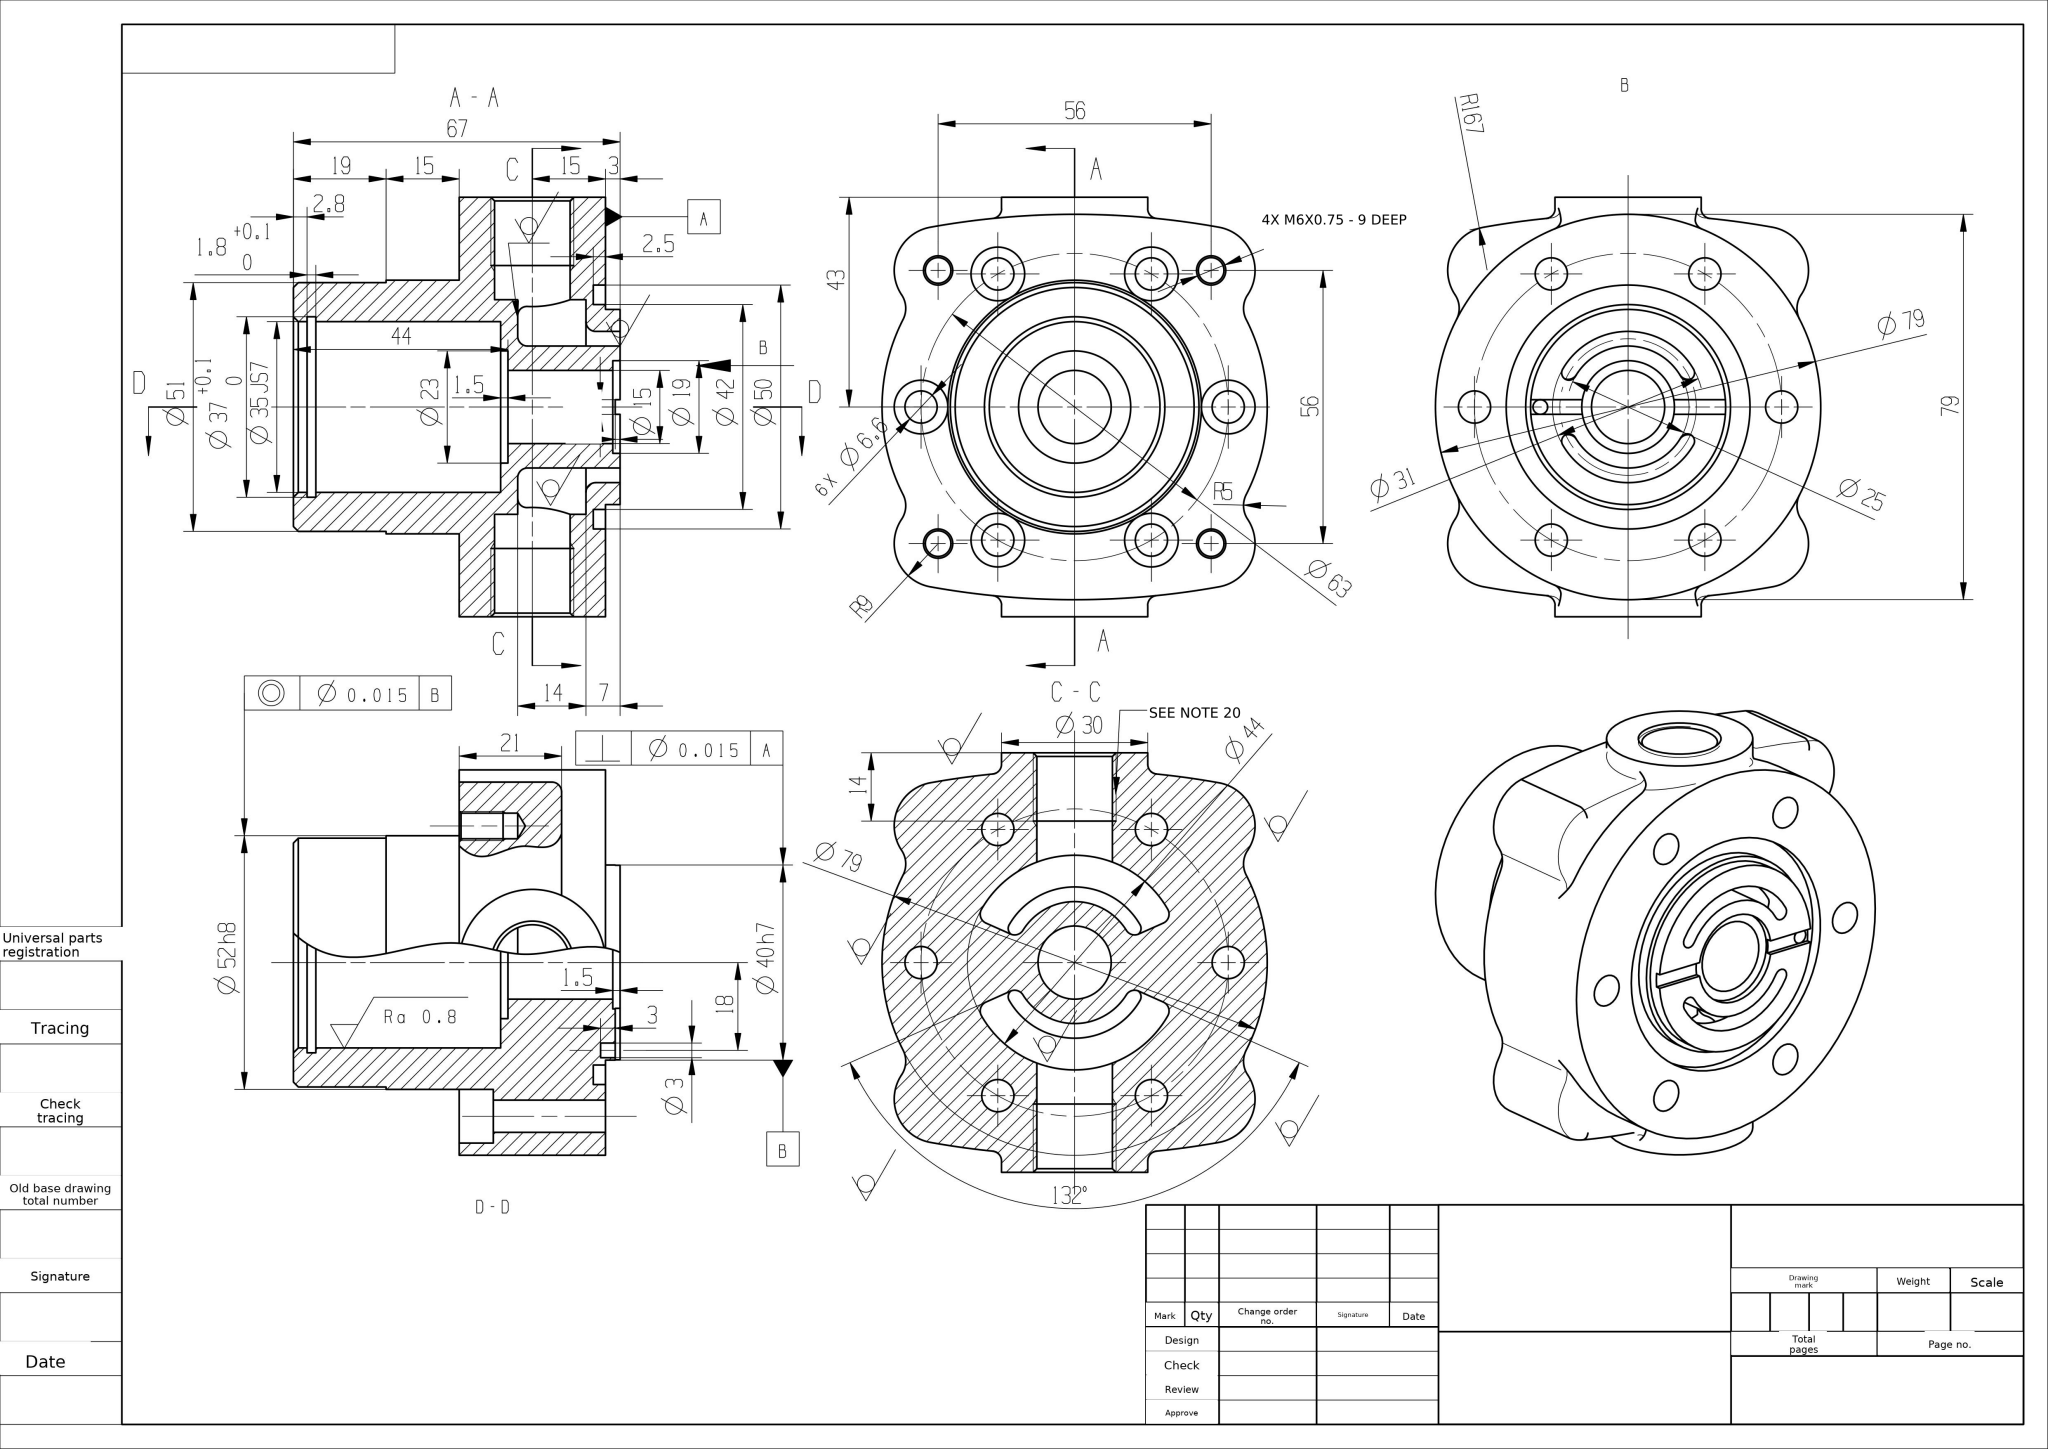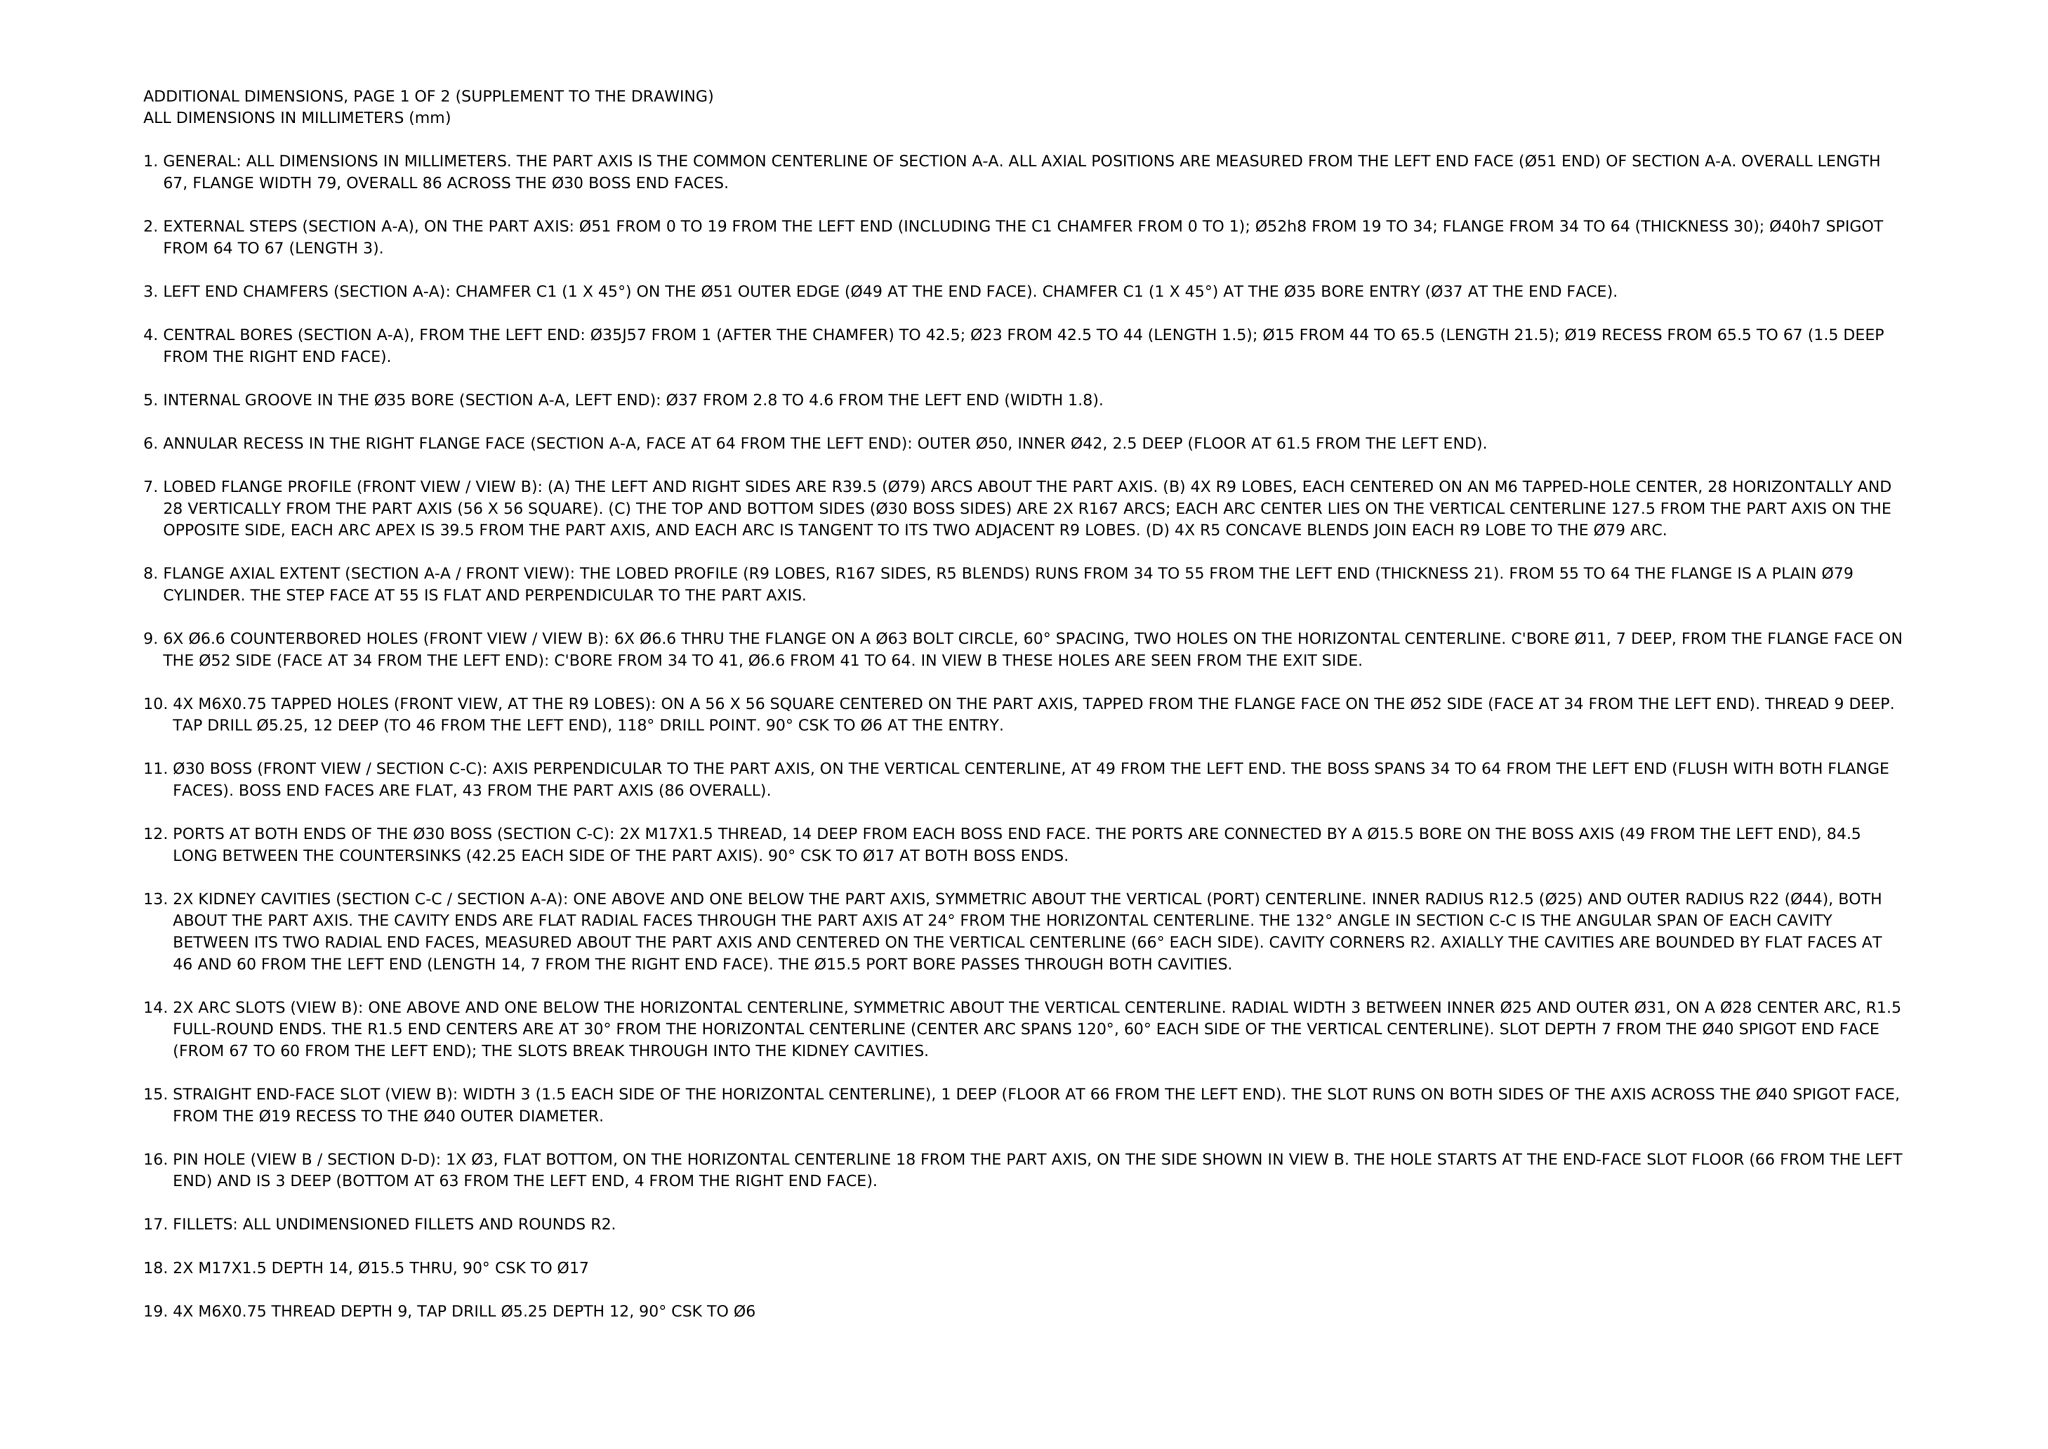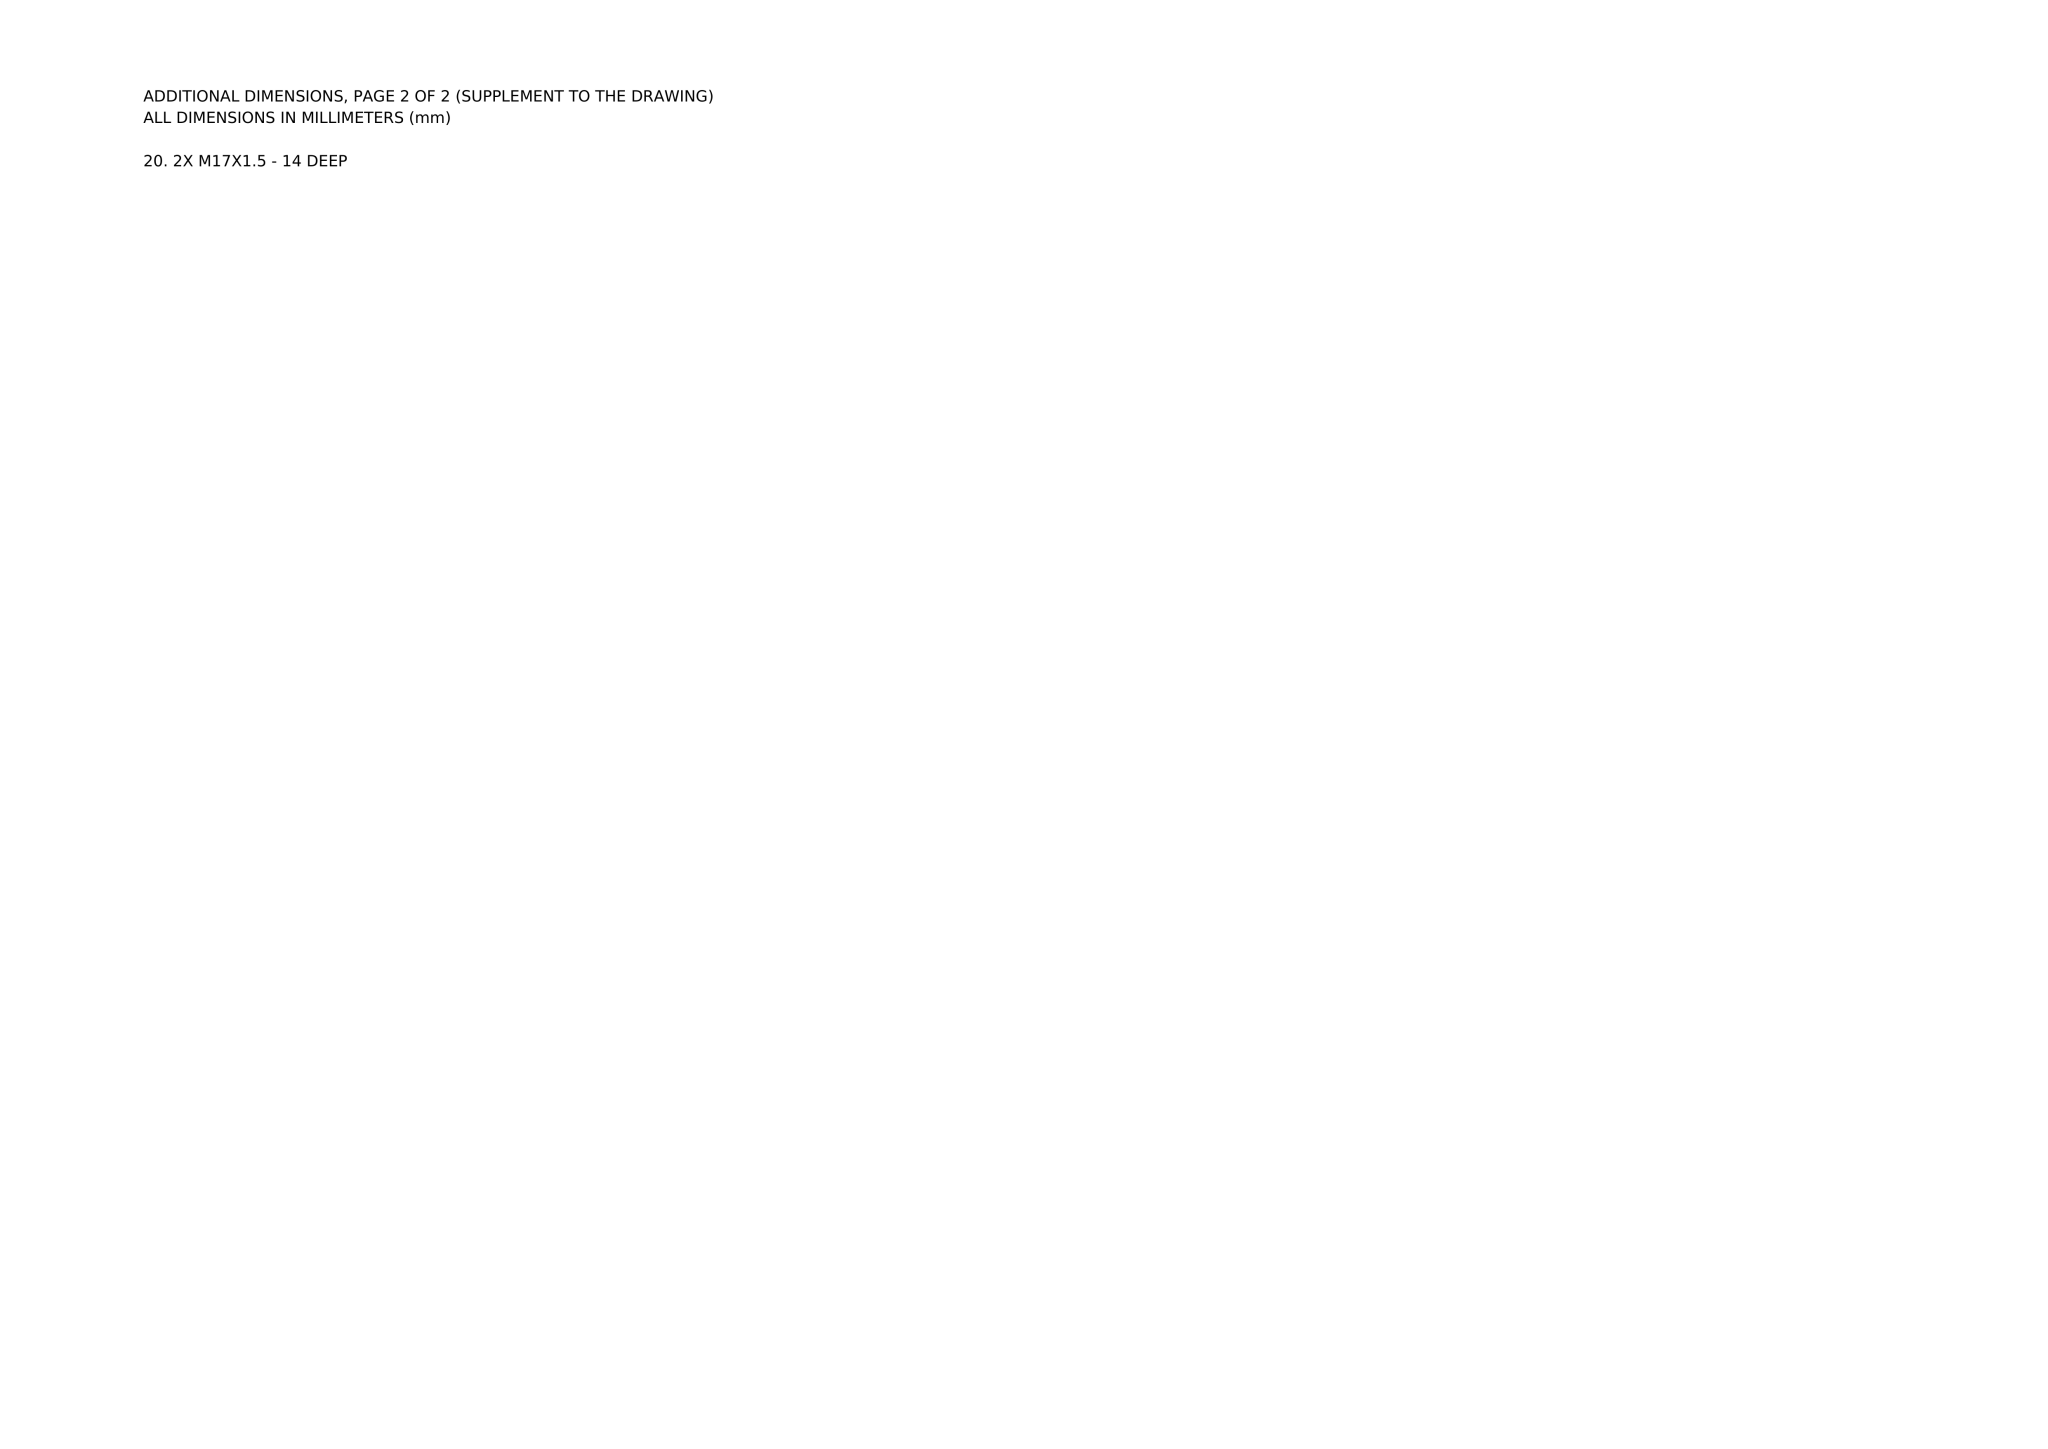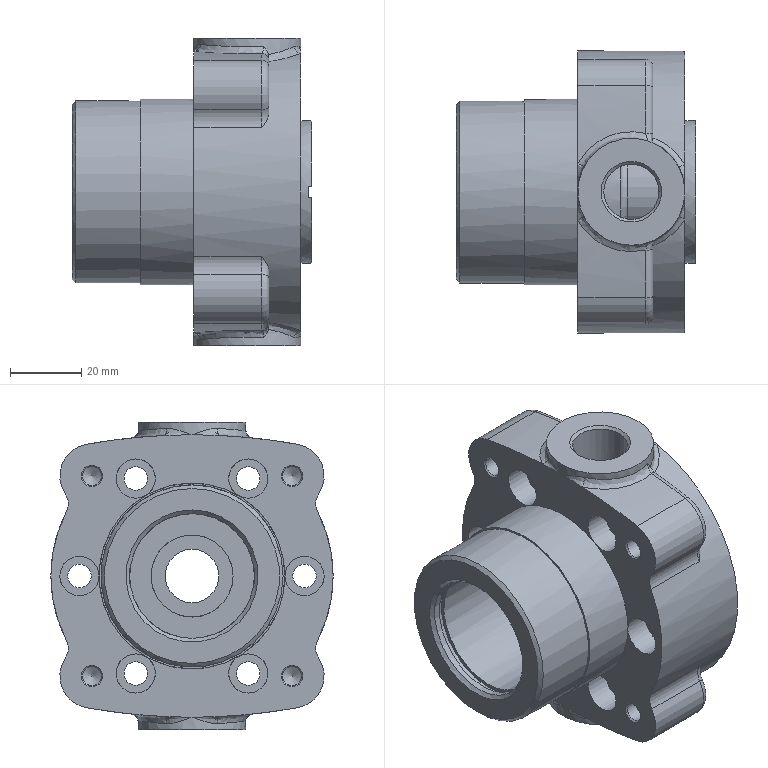Part | NX | mm | 1 solid | 179 faces | box 67 x 79 x 86 mm | volume 164747 mm3 | cylinder 70 | plane 45 | torus 24 | spline 20 | cone 12 | sphere 8 | commonest cylinder face diameters 4 x12 6.6 x6 11 x6 3 x5 44 x4 334 x4 18 x4 5.25 x4